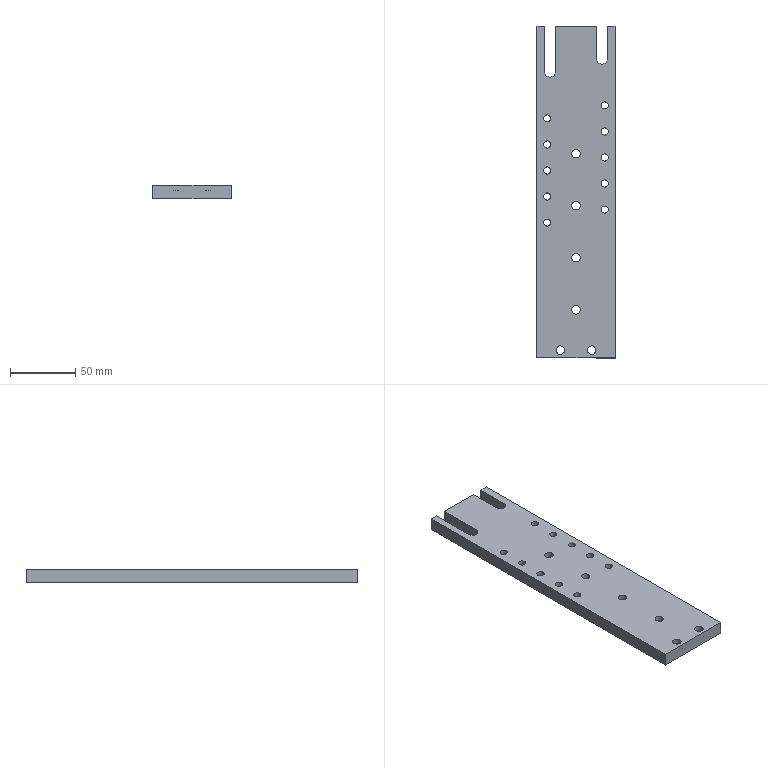Component | SolidWorks | 6GuidePlateG9.26-3 | 1 solid | 64 faces | box 60 x 255 x 10 mm | volume 140733 mm3 | cylinder 46 | plane 18 | commonest cylinder face diameters 5.5 x20 6.5 x12 11 x12 8.5 x1 8.441 x1
build123d program:
from build123d import *

# Parameters (mm, degrees)
SKETCH1_W           = 60
SKETCH1_H           = 255
BOSS_EXTRUDE1_DEPTH = 10
SKETCH2_R           = 5.5
CUT_EXTRUDE1_DEPTH  = 6.2
SKETCH3_R           = 3.25
CUT_EXTRUDE2_DEPTH  = 263.037
SKETCH5_R           = 5.5
CUT_EXTRUDE3_DEPTH  = 6
SKETCH7_R           = 3.25
CUT_EXTRUDE5_DEPTH  = 263.032
SKETCH8_R           = 2.75
CUT_EXTRUDE6_DEPTH  = 263.155
CUT_EXTRUDE7_DEPTH  = 263.155


with BuildPart() as part:
    # Sketch1 → Boss-Extrude1 (new body)
    with BuildSketch(Plane.XY):
        with Locations((30, -127.5)):
            Rectangle(SKETCH1_W, SKETCH1_H)
    extrude(amount=BOSS_EXTRUDE1_DEPTH)

    # Sketch2 → Cut-Extrude1 (cut)
    with BuildSketch(Plane.XY.offset(10)):
        with Locations((18, -249)):
            Circle(SKETCH2_R)
        with Locations((42, -249)):
            Circle(SKETCH2_R)
        with Locations((154, -249)):
            Circle(SKETCH2_R)
        with Locations((178, -249)):
            Circle(SKETCH2_R)
    extrude(amount=-CUT_EXTRUDE1_DEPTH, mode=Mode.SUBTRACT)

    # Sketch3 → Cut-Extrude2 (cut, through all)
    with BuildSketch(Plane.XY.offset(3.8)):
        with Locations((18, -249)):
            Circle(SKETCH3_R)
        with Locations((42, -249)):
            Circle(SKETCH3_R)
    extrude(amount=-CUT_EXTRUDE2_DEPTH, mode=Mode.SUBTRACT)

    # Sketch5 → Cut-Extrude3 (cut)
    with BuildSketch(Plane.XY.offset(10)):
        with Locations((30, -218)):
            Circle(SKETCH5_R)
        with Locations((30, -178)):
            Circle(SKETCH5_R)
        with Locations((30, -138)):
            Circle(SKETCH5_R)
        with Locations((30, -98)):
            Circle(SKETCH5_R)
    extrude(amount=-CUT_EXTRUDE3_DEPTH, mode=Mode.SUBTRACT)

    # Sketch7 → Cut-Extrude5 (cut, through all)
    with BuildSketch(Plane.XY.offset(4)):
        with Locations((30, -218)):
            Circle(SKETCH7_R)
        with Locations((30, -178)):
            Circle(SKETCH7_R)
        with Locations((30, -138)):
            Circle(SKETCH7_R)
        with Locations((30, -98)):
            Circle(SKETCH7_R)
    extrude(amount=-CUT_EXTRUDE5_DEPTH, mode=Mode.SUBTRACT)

    # Sketch8 → Cut-Extrude6 (cut, through all)
    with BuildSketch(Plane(origin=(0, 0, 0), x_dir=(-1, 0, 0), z_dir=(0, 0, -1))):
        with Locations((-52.042, -151)):
            Circle(SKETCH8_R)
        with Locations((-8.042, -141)):
            Circle(SKETCH8_R)
        with Locations((-52.042, -131)):
            Circle(SKETCH8_R)
        with Locations((-8.042, -121)):
            Circle(SKETCH8_R)
        with Locations((-52.042, -111)):
            Circle(SKETCH8_R)
        with Locations((-8.042, -101)):
            Circle(SKETCH8_R)
        with Locations((-52.042, -91)):
            Circle(SKETCH8_R)
        with Locations((-8.042, -81)):
            Circle(SKETCH8_R)
        with Locations((-52.042, -71)):
            Circle(SKETCH8_R)
        with Locations((-8.042, -61)):
            Circle(SKETCH8_R)
    extrude(amount=-CUT_EXTRUDE6_DEPTH, mode=Mode.SUBTRACT)

    # Sketch9 → Cut-Extrude7 (cut, through all)
    with BuildSketch(Plane(origin=(0, 0, 0), x_dir=(-1, 0, 0), z_dir=(0, 0, -1))):
        with BuildLine():
            Line((-54.25, -35), (-54.25, 6.195))
            ThreePointArc((-54.25, 6.195), (-50, 10.445), (-45.75, 6.195))
            Line((-45.75, 6.195), (-45.75, -35))
            ThreePointArc((-45.75, -35), (-50, -39.25), (-54.25, -35))
        make_face()
        with BuildLine():
            Line((-14.22, -25), (-14.22, 15.444))
            ThreePointArc((-14.22, 15.444), (-10, 19.664), (-5.78, 15.444))
            Line((-5.78, 15.444), (-5.78, -25))
            ThreePointArc((-5.78, -25), (-10, -29.22), (-14.22, -25))
        make_face()
    extrude(amount=-CUT_EXTRUDE7_DEPTH, mode=Mode.SUBTRACT)


solid = part.part

# Placed as in the assembly
solid = solid.moved(Location((150, 80, 40.5), (-180, 0, 180)))